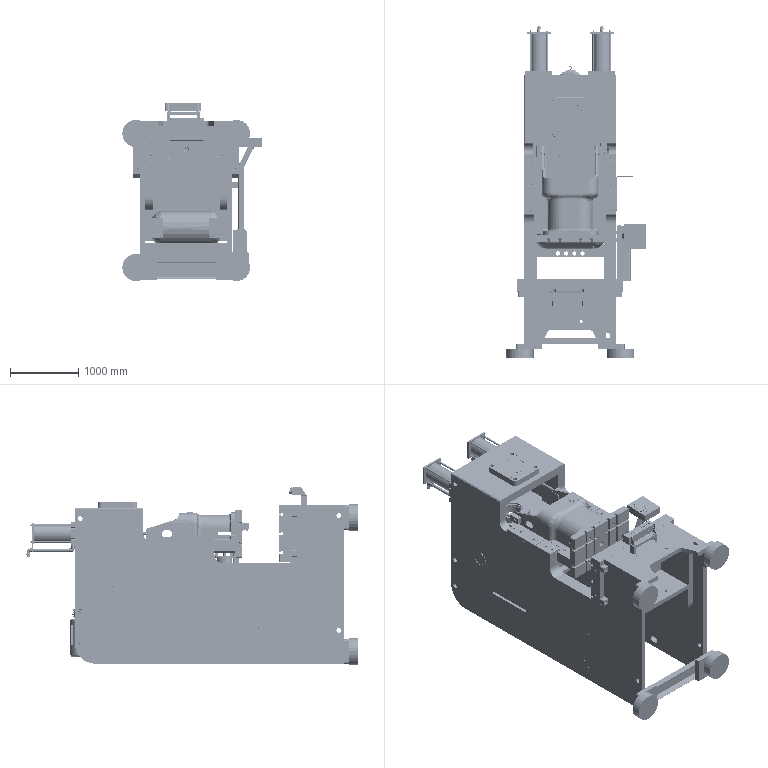Assembly | SolidWorks | mm | 147 component files | 211 solids | 10204 faces | box 2039 x 4857.81 x 2608 mm | volume 2758399652 mm3 | cylinder 4837 | plane 2910 | spline 1236 | cone 1221 | commonest cylinder face diameters 10 x1233 4 x211 6.8 x208 9 x194 6 x186 20 x126 8 x126 16 x124
Bill of materials:
200-250InverterBracket() | 1 | Plain Carbon Steel | Thin sheet bent into an L-shaped angle bracket. The larger rectangular flange has a pattern of eight through-holes. The smaller flange has no holes. The outer corners are rounded.
400ShockAbsorbingPad | 4 | Plain Carbon Steel | Plain solid cylinder shaped like a short disc or puck. It has flat parallel end faces and no visible holes or other features.
Bracket1 | 2 | Plain Carbon Steel | Flat rectangular strap or link plate with all four corners chamfered and one round through-hole near each end.
Bracket2 | 1 | Plain Carbon Steel | Formed sheet-metal cover or channel: a long top panel with walls bent down along its length and at both ends. The corners where the walls meet look mitered.
Bracket3 | 1 | Plain Carbon Steel | Gusseted angle bracket. A vertical flange with two holes and a horizontal base flange are joined by a triangular gusset wall. A short tab sticks up at the top of one edge. It looks like the mirror image of unnamed part.
Bracket4 | 1 | Plain Carbon Steel | Gusseted angle bracket: a vertical flange with two holes, a horizontal base flange, and a triangular gusset side wall. A narrow tab sticks up at the top edge. It looks like the mirror image of unnamed part.
ButtonStationBase1 | 1 | Plain Carbon Steel | Long L-shaped sheet-metal angle. Both legs have short return lips. The vertical leg has notched edges and several holes, including one large round hole and a smaller hole surrounded by four small holes.
ButtonStationTopCover | 1 | Plain Carbon Steel | Inverted-U sheet-metal channel or bridge. A long flat top has a row of round holes, and the two end legs are tapered (trapezoidal). A long front face carries a further row of holes.
Hinge1 | 2 | Plain Carbon Steel | Hinge-leaf-like plate: a flat rectangular leaf with a hollow cylindrical knuckle at each end of one edge and a rectangular gap between the two knuckles.
Hinge2 | 2 | Plain Carbon Steel | Hinge-leaf-like plate: a flat rectangular leaf with a single hollow cylindrical knuckle in the middle of one long edge.
Two-HandButtonGuardRing | 2 | Plain Carbon Steel | Thin strip bent into a U shape: a semicircular bottom with two straight parallel legs. The legs have rounded free corners, and the side view shows a tapered outline.
YC1-200-01-11BodySideCover | 1 | Plain Carbon Steel | Thin flat circular disc with six round through-holes spaced evenly on a circle near the outer edge.
YC1-200-03-0202UpperWorkbench# | 1 | Plain Carbon Steel | Thick rectangular plate with small corner chamfers. One large face has two parallel T-slots running lengthwise and four T-slots running across it. It has a central through-hole and a pattern of smaller holes.
YC1-250-01-01MachineBody#_Default_ByMachining | 1 | Plain Carbon Steel | Large open box-like frame or housing. Its side walls have a stepped top profile with a cutout and a large rounded corner at the bottom. It has a raised upper block containing two large circular bores, rectangular openings in the faces, cross members and many small holes. The ends carry mounting tabs, each with several holes.
YC1-250-02-06RearCrankshaftBearing | 1 | Plain Carbon Steel | Thin-walled cylindrical sleeve (a short tube). It has a small outward lip at one end, a slight chamfer or taper at the other end, and a groove or line inside the bore.
YC1-250-03-07RearGuideLiner | 4 | Plain Carbon Steel | Rectangular block plate. One face has a shallow serpentine groove that winds back and forth. It has four countersunk corner holes, a countersunk central hole and a small hole at one end of the groove.
YC1-250-03-08LeftGuideLiner | 2 | Plain Carbon Steel | Rectangular plate. One face has a shallow serpentine groove forming U-shaped loops. It has four countersunk corner holes, a countersunk central hole and a small hole on one groove leg.
YC1-250-01-04Workbench | 1 | Plain Carbon Steel | Thick rectangular plate with a central rectangular window that has rounded corners. It has holes through the face, small holes and T-slot profiles on one end face, and a notch or step along one long edge.
YC1-250-01-05BodyRearCover | 1 | Plain Carbon Steel | Flat circular flange plate with a central through-hole. A raised circular boss with an external groove sits on it. The outer rim has a ring of small holes.
YC1-250-01-07SafetyGuard | 1 | Plain Carbon Steel | Thin flat rectangular sheet with a regular grid of small perforations. It has a few edge holes or slots around the border.
YC1-250-02-02CrankshaftBearingSeat | 1 | Plain Carbon Steel | Square flange with rounded corners. It has four corner through-holes, two smaller diagonal holes and a large central bore. A stepped cylindrical spigot sticks out from the underside.
YC1-250-02-05FrontCrankshaftBearing | 1 | Plain Carbon Steel | Flanged cylindrical sleeve: a thin tube with a wider flat flange at one end and a chamfer at the other end.
BearingGBNU2319E_RollingBearingsNU2319EGB283-94 | 1 | Plain Carbon Steel | Annular body that looks like a rolling-element bearing: an outer ring, an inner ring and a ring of round elements between them.
YC1-250-02-03FrontDriveBearingSeat | 1 | Plain Carbon Steel | Circular cap or plug-like disk. It has a wide flat top flange and a smaller-diameter cylindrical spigot below with an external groove and a chamfered lower edge. The flange has a ring of holes.
YC1-250-02-23FrontDriveBearingSeatGland | 1 | Plain Carbon Steel | Thin flat annular ring with a large central opening and six small through holes evenly spaced on a bolt circle.
YC1-250-02-12RearRetainingRing | 1 | Plain Carbon Steel | Short thin-walled cylindrical ring with an internal step or lip near one end.
YC1-250-02-20CrankshaftFrontEndAdjustmentCover | 1 | Plain Carbon Steel | Solid circular disc with eight through holes evenly spaced on a bolt circle and no central opening.
YC1-250-02-21CrankshaftEndCover | 1 | Plain Carbon Steel | Very thin solid circular disc with six small holes evenly spaced close to the perimeter.
TECOFixedSpeed25HP_4P | 1 | Plain Carbon Steel | Cylindrical housing with rounded end caps, one projecting shaft, axial external ribs, side mounting feet/brackets with holes, a lifting ring on top, and a side-mounted box. Overall it looks like a foot-mounted electric motor.
YC1-200-02-29AdjustmentScrew | 4 | Plain Carbon Steel | Cylindrical sleeve with an axial through bore and a smaller hexagonal section at one end.
YC1-250-02-1801Pulley | 1 | Plain Carbon Steel | Multi-groove sheave/pulley with five circumferential V-shaped grooves between six rims, a recessed face, a central hub with a keyed bore, and two small holes in the web.
YC1-250-02-25MotorShaftEndCover | 1 | Plain Carbon Steel | Plain flat round washer-like disc with a single central through hole.
YC1-250-02-28MotorSeat | 1 | Plain Carbon Steel | Thin rectangular plate with four larger corner holes, six small holes in two columns, a V-shaped notch on one short edge, and small chamfered corners.
BearingGB-6309_RollingBearings6309GB276-94 | 2 | Plain Carbon Steel | Shape that looks like a deep-groove ball bearing: concentric outer and inner rings with one row of balls between them, and no visible cage or shields.
JinsongDigitalDisplayXSQ-1 | 1 | Plain Carbon Steel | Rectangular box-shaped enclosure with a wider top flange plate that has four corner holes, rounded lower edges, and a stepped cylindrical pin projecting from the bottom. The top face has raised or engraved characters inside a rounded rectangular outline.
Oil-ImpregnatedCopper | 1 | Plain Carbon Steel | Cylindrical tube/sleeve with a fairly thick wall, chamfered ends, and many radial round through holes arranged in axial columns of three around the circumference.
YC1-110-03-38LargeSprocketGland | 1 | Plain Carbon Steel | Flat circular disc with a single concentric through-hole; washer-like annulus.
YC1-160-03-22WormGland | 1 | Plain Carbon Steel | Round flanged annular housing: a thin outer flange with six through-holes around it and a raised cylindrical boss with a stepped central bore and a groove around its outside.
YC1-160-03-32LargeSprocket | 1 | Plain Carbon Steel | Thin circular plate with six round holes evenly spaced around the center and a two-step central hub with a keyed through-bore.
YC1-160-03-35Oil-ImpregnatedCopperSeat | 1 | Plain Carbon Steel | Thick-walled cylindrical sleeve/bushing with a large through-bore, a narrow external groove near one end, and chamfered outer edges.
YC1-200-03-33SmallSprocket | 1 | Plain Carbon Steel | Flanged bushing: a wide chamfered disc flange on top of a cylindrical shank with a reduced-diameter neck/undercut, and a central bore with a keyway.
YC1-200-03-34DiscMotorSeat | 1 | Plain Carbon Steel | Thin square plate with chamfered corners, a large central circular opening, four elongated slots near the corners and four small round holes.
YC1-200-03-39SmallSprocketGland | 1 | Plain Carbon Steel | Solid cylinder with a small concentric through-hole: a thick spacer- or roller-like body.
YC1-250-03-01Slider | 1 | Plain Carbon Steel | Complex housing/bracket: a rectangular base with long rails, a rounded tunnel-like central shell, upright end walls with rectangular windows and holes, and sloped side lugs with holes.
YC1-250-03-03WormGear | 1 | Plain Carbon Steel | Toothed ring gear with external teeth, a large central bore with one keyway, and short radial marks/notches on one face.
YC1-250-03-04Worm | 1 | Plain Carbon Steel | Stepped shaft with an integral helical threaded/worm section partway along its length, several shoulder diameters, and a slotted or flatted end.
YC1-250-03-18BallHeadGland | 1 | Plain Carbon Steel | Flanged annular cover/adapter: a circular flange with a ring of through-holes and a raised chamfered cylindrical spigot around a large central bore.
YC1-250-03-23HydraulicCylinderPressurePlate | 1 | Plain Carbon Steel | Long flat rectangular bar/plate with chamfered corners, a large central hole, four small holes around it, and two holes at each end.
YC1-250-03-27BalancerConnectingPin | 2 | Plain Carbon Steel | Stepped solid cylinder: a larger-diameter body, a thin raised collar, and a smaller-diameter coaxial spigot with a chamfered end and a small central axial hole.
YC1-250-03-37Gland | 2 | Plain Carbon Steel | Thin flat circular disc with a single small central through hole, washer-like in form.
YC1-T-FCD-X8 | 1 | Plain Carbon Steel | Very thin flat annular ring (shim- or washer-like) with a large central hole.
YPE1100S2-4Z | 1 | Plain Carbon Steel | Round cup-shaped housing with a wide circular flange at the top and four equally spaced holes in the flange. The flange face has a raised circular step. A slender central shaft sticks out from it, and the base is rounded with a slight bottom boss.
YC1-250-03-06FrontGuideLiner | 2 | Plain Carbon Steel | Long, thin, flat rectangular bar with a row of small through holes along its length. The holes alternate between the two long edges, and there are extra hole clusters at each end.
YC1-250-03-10LeftPressurePlate | 1 | Plain Carbon Steel | Rectangular flat bar with a row of through holes along its length: larger holes plus two smaller holes. It has a narrow transverse groove across the top face, chamfered top edges, and a stepped profile on the underside.
YC1-250-03-11RightPressurePlate | 1 | Plain Carbon Steel | Rectangular flat bar similar to unnamed part. It has the same set of larger and smaller through holes, a transverse groove across the top face, chamfered top edges, and a stepped underside on the opposite side.
YC1-250-03-09RightGuideLiner | 2 | Plain Carbon Steel | Thin rectangular plate with six round through holes: one near each corner and two more along the horizontal centerline, placed off-center.
YC1-250-03-12AdjustmentPlate | 2 | Plain Carbon Steel | Thick rectangular block-plate. The main face has four larger corner through holes, each with a small adjacent hole, plus a small central hole. There are also two small holes on one long edge face.
GBHexNutM20_GB_FASTENER_NUT_SNC1M16-N | 8 | Plain Carbon Steel | Elongated hexagonal prism with a round coaxial through bore and chamfered or crowned ends, like a long hex nut or coupling-nut form.
GBSpringWasherM20_GB_FASTENER_WASHER_SW16 | 8 | Plain Carbon Steel | Flat annular ring with a rectangular-section rim and a single radial split, resembling a split-washer form.
Rc11-4Elbow | 4 | Plain Carbon Steel | Hollow tubular 90-degree elbow. Two straight cylindrical legs, each with an open end, are joined by a smoothly curved bend.
Rc11-4StraightInternalConnection | 4 | Plain Carbon Steel | Bushing-like part: a hollow cylinder with a through bore and a hexagonal collar around its middle.
YC1-250-04-01Base#16673 | 2 | Plain Carbon Steel | Rectangular plate with four open-ended U-slots, a central hole, a smaller hole, and a thin circular boss on one face.
YC1-250-04-02TopCover#16673(1) | 2 | Plain Carbon Steel | Rectangular plate with a large central hole, six smaller holes around the edge, a small hole off-center, and a shallow circular raised pilot on one face.
YC1-250-04-04CylinderBarrel#16673 | 2 | Plain Carbon Steel | Short, thin-walled, open-ended cylindrical tube.
YC1-250-04-05#16673Piston | 2 | Plain Carbon Steel | Disc or wheel with a central bore and a circumferential groove around the rim, pulley-like in shape.
YC1-250-04-06TieRodAxis#16673 | 2 | Plain Carbon Steel | Long, slender cylindrical shaft with a reduced-diameter step at each end and small cross holes near both ends.
YC1-250-04-07TieRodSeat | 2 | Plain Carbon Steel | Rectangular block with an arch-shaped (U-shaped) slot through its thickness, open at the bottom, and a small through hole beside the slot.
YC1-250-04-08Washer | 2 | Plain Carbon Steel | Flat annular ring, washer-like in shape.
YC1-250-04-09Cover | 2 | Plain Carbon Steel | Thin, flat circular disc with two small through holes on opposite sides.
YC1-250-04-10Double-endedScrew#16673 | 8 | Plain Carbon Steel | Long, slender solid rod with a reduced-diameter step at one end.
YC1-250-04-11Standpipe#16673 | 2 | Plain Carbon Steel | Long, thin-walled, open-ended tube with slightly tapered or chamfered ends.
YC1-250-04-12#16673PipeSeat | 2 | Plain Carbon Steel | Rectangular block split by a thin gap into a larger upper portion and a smaller lower portion, with a circular bore centered on the split line, clamp-like in shape.
YC1-250-04-13#16673Sleeve | 8 | Plain Carbon Steel | Straight thin-walled round tube with plain, square-cut ends.
YC1-250-06-01AirTank | 1 | Plain Carbon Steel | Horizontal cylindrical vessel with domed ends, two L-section mounting brackets along one side, and several small cylindrical nozzles or bosses on the shell.
YC1-250-06-03AirTankFixingSeat | 2 | Plain Carbon Steel | Sheet-metal angle bracket made of two plates at right angles, braced by two tapered triangular gusset ribs. The short flange has two oblong slots and the far edge of the long leg has two open-ended slots.
YC1-25-01-08OilHoleCover | 1 | Plain Carbon Steel | Thin flat circular disc with two small through-holes, diametrically opposite each other near the edge.
80-315ControlPanel | 1 | Plain Carbon Steel | Rectangular block with a pattern of circular holes or recesses on the top face, plus a shallow rectangular recess or step outline across part of that face.
80-315ElectricalBox | 1 | Plain Carbon Steel | Shallow rectangular box-like housing with rounded edges, a square opening in the top face, and four small bent mounting tabs on two opposite sides.
YC1-160BoxBaffleT | 1 | Plain Carbon Steel | Flat square plate frame with a large central square opening that has rounded inner corners.
YC1-160OperationStationBaffleT | 1 | Plain Carbon Steel | Thin flat rectangular plate with four corner through-holes and a central rectangular cutout with small corner radii.
YC1-160SmallBracketT | 1 | Plain Carbon Steel | Formed sheet-metal hat-section (omega) bracket: a central U-shaped channel with two outward flanges, each flange having two oblong slots.
YC1-250OperationStationConnectingArmT_Default_ByMachining | 1 | Plain Carbon Steel | Square hollow tube with rounded corners and a single dog-leg offset bend near one end, ending in a short straight section that appears to be a sleeve or stepped end.
Mates: